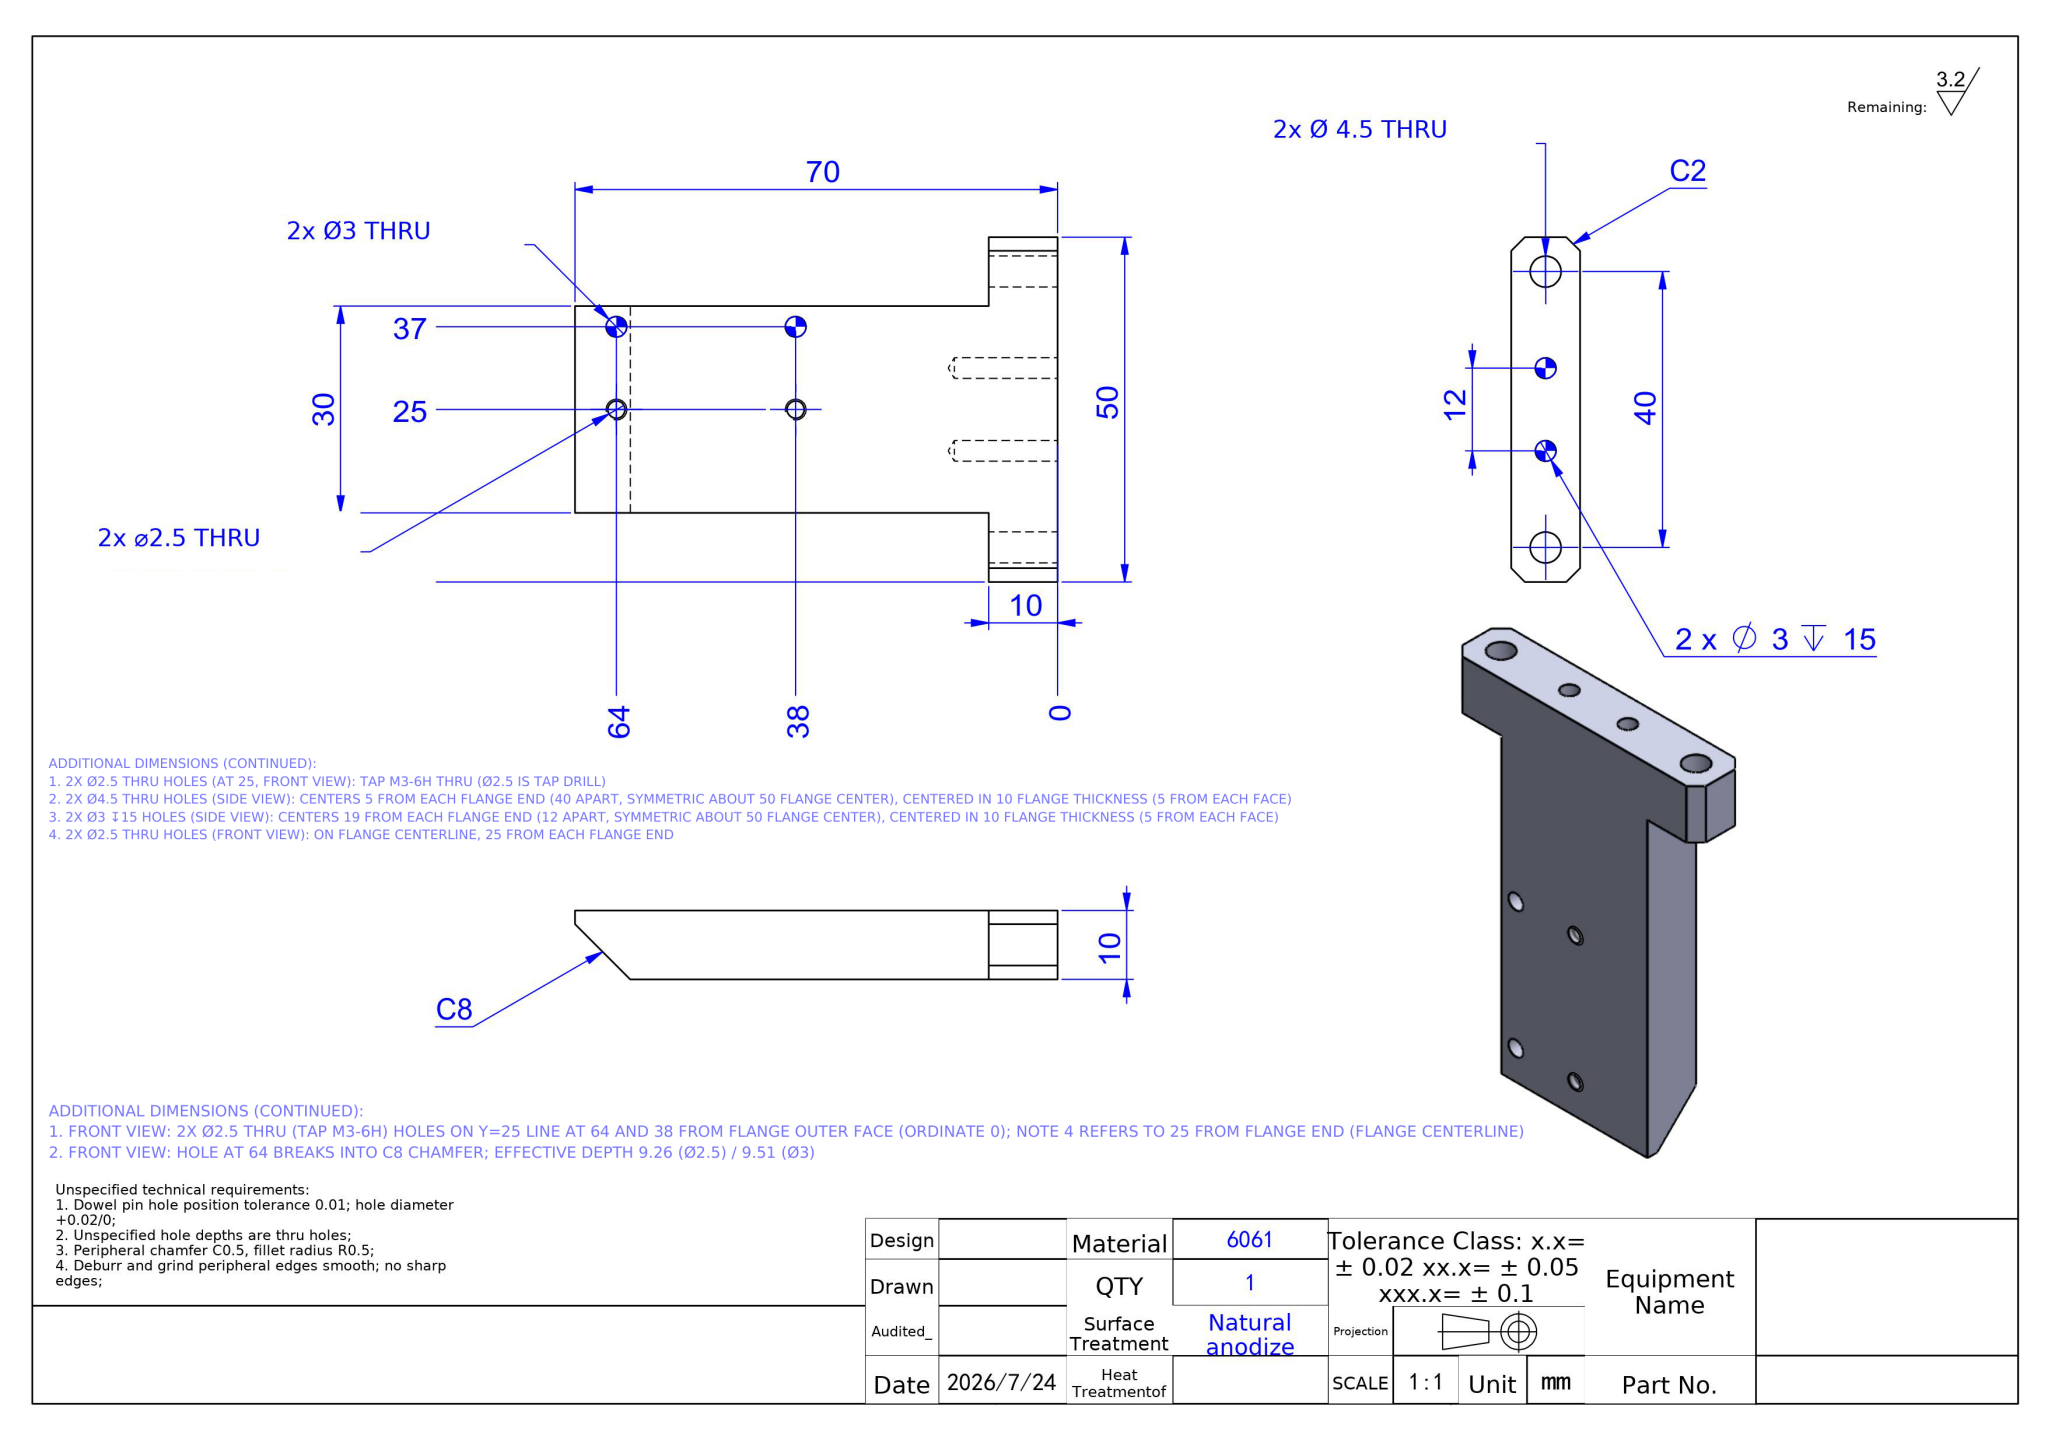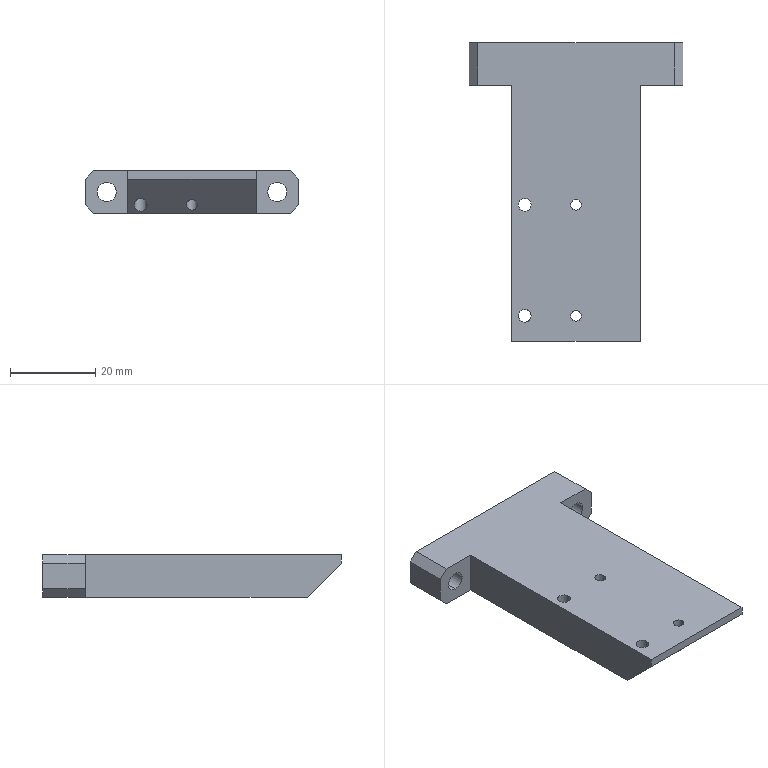Part | NX | mm | 1 solid | 35 faces | box 50 x 70 x 10 mm | volume 21210 mm3 | cylinder 16 | plane 15 | cone 4 | commonest cylinder face diameters 3 x8 2.5 x4 4.5 x4